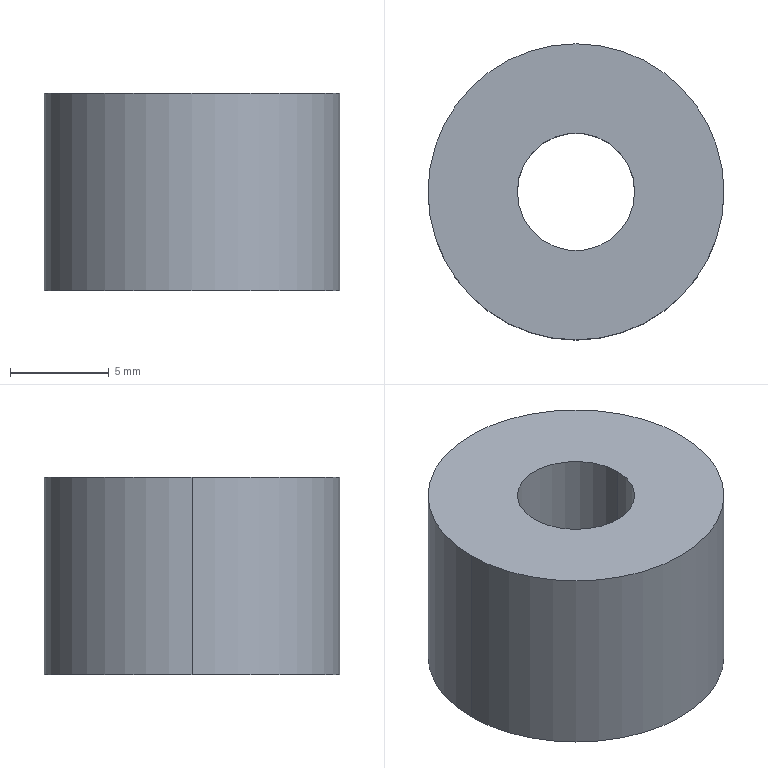Component | SolidWorks | SmallWheel-1 | 1 solid | 6 faces | box 15 x 15 x 10 mm | volume 1489 mm3 | cylinder 4 | plane 2 | commonest cylinder face diameters 5.952 x2 15 x2
build123d program:
from build123d import *

# Parameters (mm, degrees)
SKETCH1_R           = 7.5
SKETCH1_R_2         = 2.976
BOSS_EXTRUDE1_DEPTH = 10


with BuildPart() as part:
    # Sketch1 → Boss-Extrude1 (new body)
    with BuildSketch(Plane.XY):
        with Locations((59.88, -20)):
            Circle(SKETCH1_R)
        with Locations((59.88, -20)):
            Circle(SKETCH1_R_2, mode=Mode.SUBTRACT)
    extrude(amount=-BOSS_EXTRUDE1_DEPTH)


solid = part.part

# Placed as in the assembly
solid = solid.moved(Location((-11.374, -44.609, -195), (0, 0, 0)))
STEP:
#1=COLOUR_RGB('',0.7922,0.8196,0.9333);
#2=FILL_AREA_STYLE_COLOUR('',#1);
#3=FILL_AREA_STYLE('',(#2));
#4=SURFACE_STYLE_FILL_AREA(#3);
#5=SURFACE_SIDE_STYLE('',(#4));
#6=SURFACE_STYLE_USAGE(.BOTH.,#5);
#7=PRESENTATION_STYLE_ASSIGNMENT((#6));
#8=CARTESIAN_POINT('',(1.793,-2.544,-8.071));
#9=VERTEX_POINT('',#8);
#10=CARTESIAN_POINT('',(2.027,-2.544,-8.071));
#11=VERTEX_POINT('',#10);
#12=CARTESIAN_POINT('',(1.91,-2.544,-8.071));
#13=DIRECTION('',(0.,0.,1.));
#14=DIRECTION('',(1.,0.,0.));
#15=AXIS2_PLACEMENT_3D('',#12,#13,#14);
#16=CIRCLE('',#15,0.1172);
#17=EDGE_CURVE('',#9,#11,#16,.T.);
#18=ORIENTED_EDGE('',*,*,#17,.F.);
#19=CARTESIAN_POINT('',(1.793,-2.544,-7.677));
#20=VERTEX_POINT('',#19);
#21=CARTESIAN_POINT('',(1.793,-2.544,-8.071));
#22=DIRECTION('',(0.,0.,1.));
#23=VECTOR('',#22,39.37);
#24=LINE('',#21,#23);
#25=EDGE_CURVE('',#9,#20,#24,.T.);
#26=ORIENTED_EDGE('',*,*,#25,.T.);
#27=CARTESIAN_POINT('',(2.027,-2.544,-7.677));
#28=VERTEX_POINT('',#27);
#29=CARTESIAN_POINT('',(1.91,-2.544,-7.677));
#30=DIRECTION('',(0.,0.,1.));
#31=DIRECTION('',(1.,0.,0.));
#32=AXIS2_PLACEMENT_3D('',#29,#30,#31);
#33=CIRCLE('',#32,0.1172);
#34=EDGE_CURVE('',#20,#28,#33,.T.);
#35=ORIENTED_EDGE('',*,*,#34,.T.);
#36=CARTESIAN_POINT('',(2.027,-2.544,-8.071));
#37=DIRECTION('',(0.,0.,1.));
#38=VECTOR('',#37,39.37);
#39=LINE('',#36,#38);
#40=EDGE_CURVE('',#11,#28,#39,.T.);
#41=ORIENTED_EDGE('',*,*,#40,.F.);
#42=EDGE_LOOP('',(#18,#26,#35,#41));
#43=FACE_OUTER_BOUND('',#42,.T.);
#44=CARTESIAN_POINT('',(1.91,-2.544,-8.071));
#45=DIRECTION('',(0.,0.,1.));
#46=DIRECTION('',(1.,0.,0.));
#47=AXIS2_PLACEMENT_3D('',#44,#45,#46);
#48=CYLINDRICAL_SURFACE('',#47,0.1172);
#49=ADVANCED_FACE('',(#43),#48,.F.);
#50=CARTESIAN_POINT('',(2.205,-2.544,-8.071));
#51=VERTEX_POINT('',#50);
#52=CARTESIAN_POINT('',(1.614,-2.544,-8.071));
#53=VERTEX_POINT('',#52);
#54=CARTESIAN_POINT('',(1.91,-2.544,-8.071));
#55=DIRECTION('',(0.,0.,1.));
#56=DIRECTION('',(1.,0.,0.));
#57=AXIS2_PLACEMENT_3D('',#54,#55,#56);
#58=CIRCLE('',#57,0.2953);
#59=EDGE_CURVE('',#51,#53,#58,.T.);
#60=ORIENTED_EDGE('',*,*,#59,.T.);
#61=CARTESIAN_POINT('',(1.614,-2.544,-7.677));
#62=VERTEX_POINT('',#61);
#63=CARTESIAN_POINT('',(1.614,-2.544,-8.071));
#64=DIRECTION('',(0.,0.,1.));
#65=VECTOR('',#64,39.37);
#66=LINE('',#63,#65);
#67=EDGE_CURVE('',#53,#62,#66,.T.);
#68=ORIENTED_EDGE('',*,*,#67,.T.);
#69=CARTESIAN_POINT('',(2.205,-2.544,-7.677));
#70=VERTEX_POINT('',#69);
#71=CARTESIAN_POINT('',(1.91,-2.544,-7.677));
#72=DIRECTION('',(0.,0.,1.));
#73=DIRECTION('',(1.,0.,0.));
#74=AXIS2_PLACEMENT_3D('',#71,#72,#73);
#75=CIRCLE('',#74,0.2953);
#76=EDGE_CURVE('',#70,#62,#75,.T.);
#77=ORIENTED_EDGE('',*,*,#76,.F.);
#78=CARTESIAN_POINT('',(2.205,-2.544,-8.071));
#79=DIRECTION('',(0.,0.,1.));
#80=VECTOR('',#79,39.37);
#81=LINE('',#78,#80);
#82=EDGE_CURVE('',#51,#70,#81,.T.);
#83=ORIENTED_EDGE('',*,*,#82,.F.);
#84=EDGE_LOOP('',(#60,#68,#77,#83));
#85=FACE_OUTER_BOUND('',#84,.T.);
#86=CARTESIAN_POINT('',(1.91,-2.544,-8.071));
#87=DIRECTION('',(0.,0.,1.));
#88=DIRECTION('',(1.,0.,0.));
#89=AXIS2_PLACEMENT_3D('',#86,#87,#88);
#90=CYLINDRICAL_SURFACE('',#89,0.2953);
#91=ADVANCED_FACE('',(#85),#90,.T.);
#92=ORIENTED_EDGE('',*,*,#67,.F.);
#93=CARTESIAN_POINT('',(1.91,-2.544,-8.071));
#94=DIRECTION('',(0.,0.,1.));
#95=DIRECTION('',(1.,0.,0.));
#96=AXIS2_PLACEMENT_3D('',#93,#94,#95);
#97=CIRCLE('',#96,0.2953);
#98=EDGE_CURVE('',#53,#51,#97,.T.);
#99=ORIENTED_EDGE('',*,*,#98,.T.);
#100=ORIENTED_EDGE('',*,*,#82,.T.);
#101=CARTESIAN_POINT('',(1.91,-2.544,-7.677));
#102=DIRECTION('',(0.,0.,1.));
#103=DIRECTION('',(1.,0.,0.));
#104=AXIS2_PLACEMENT_3D('',#101,#102,#103);
#105=CIRCLE('',#104,0.2953);
#106=EDGE_CURVE('',#62,#70,#105,.T.);
#107=ORIENTED_EDGE('',*,*,#106,.F.);
#108=EDGE_LOOP('',(#92,#99,#100,#107));
#109=FACE_OUTER_BOUND('',#108,.T.);
#110=CARTESIAN_POINT('',(1.91,-2.544,-8.071));
#111=DIRECTION('',(0.,0.,1.));
#112=DIRECTION('',(1.,0.,0.));
#113=AXIS2_PLACEMENT_3D('',#110,#111,#112);
#114=CYLINDRICAL_SURFACE('',#113,0.2953);
#115=ADVANCED_FACE('',(#109),#114,.T.);
#116=CARTESIAN_POINT('',(1.91,-2.544,-8.071));
#117=DIRECTION('',(0.,0.,1.));
#118=DIRECTION('',(1.,0.,0.));
#119=AXIS2_PLACEMENT_3D('',#116,#117,#118);
#120=CIRCLE('',#119,0.1172);
#121=EDGE_CURVE('',#11,#9,#120,.T.);
#122=ORIENTED_EDGE('',*,*,#121,.T.);
#123=ORIENTED_EDGE('',*,*,#17,.T.);
#124=EDGE_LOOP('',(#122,#123));
#125=FACE_BOUND('',#124,.T.);
#126=ORIENTED_EDGE('',*,*,#59,.F.);
#127=ORIENTED_EDGE('',*,*,#98,.F.);
#128=EDGE_LOOP('',(#126,#127));
#129=FACE_OUTER_BOUND('',#128,.T.);
#130=CARTESIAN_POINT('',(1.91,-2.544,-8.071));
#131=DIRECTION('',(0.,0.,1.));
#132=DIRECTION('',(1.,0.,0.));
#133=AXIS2_PLACEMENT_3D('',#130,#131,#132);
#134=PLANE('',#133);
#135=ADVANCED_FACE('',(#125,#129),#134,.F.);
#136=CARTESIAN_POINT('',(1.91,-2.544,-7.677));
#137=DIRECTION('',(0.,0.,1.));
#138=DIRECTION('',(1.,0.,0.));
#139=AXIS2_PLACEMENT_3D('',#136,#137,#138);
#140=CIRCLE('',#139,0.1172);
#141=EDGE_CURVE('',#28,#20,#140,.T.);
#142=ORIENTED_EDGE('',*,*,#141,.F.);
#143=ORIENTED_EDGE('',*,*,#34,.F.);
#144=EDGE_LOOP('',(#142,#143));
#145=FACE_BOUND('',#144,.T.);
#146=ORIENTED_EDGE('',*,*,#76,.T.);
#147=ORIENTED_EDGE('',*,*,#106,.T.);
#148=EDGE_LOOP('',(#146,#147));
#149=FACE_OUTER_BOUND('',#148,.T.);
#150=CARTESIAN_POINT('',(1.91,-2.544,-7.677));
#151=DIRECTION('',(0.,0.,1.));
#152=DIRECTION('',(1.,0.,0.));
#153=AXIS2_PLACEMENT_3D('',#150,#151,#152);
#154=PLANE('',#153);
#155=ADVANCED_FACE('',(#145,#149),#154,.T.);
#156=ORIENTED_EDGE('',*,*,#25,.F.);
#157=ORIENTED_EDGE('',*,*,#121,.F.);
#158=ORIENTED_EDGE('',*,*,#40,.T.);
#159=ORIENTED_EDGE('',*,*,#141,.T.);
#160=EDGE_LOOP('',(#156,#157,#158,#159));
#161=FACE_OUTER_BOUND('',#160,.T.);
#162=CARTESIAN_POINT('',(1.91,-2.544,-8.071));
#163=DIRECTION('',(0.,0.,1.));
#164=DIRECTION('',(1.,0.,0.));
#165=AXIS2_PLACEMENT_3D('',#162,#163,#164);
#166=CYLINDRICAL_SURFACE('',#165,0.1172);
#167=ADVANCED_FACE('',(#161),#166,.F.);
#168=CLOSED_SHELL('',(#49,#91,#115,#135,#155,#167));
#169=MANIFOLD_SOLID_BREP('',#168);
#170=STYLED_ITEM('',(#7),#169);
#171=(LENGTH_UNIT()NAMED_UNIT(*)SI_UNIT($,.METRE.));
#172=LENGTH_MEASURE_WITH_UNIT(LENGTH_MEASURE(0.0254),#171);
#173=DIMENSIONAL_EXPONENTS(1.,0.,0.,0.,0.,0.,0.);
#174=(CONVERSION_BASED_UNIT('',#172)LENGTH_UNIT()NAMED_UNIT(#173));
#175=UNCERTAINTY_MEASURE_WITH_UNIT(LENGTH_MEASURE(0.00001),#174,'','');
#176=(NAMED_UNIT(*)PLANE_ANGLE_UNIT()SI_UNIT($,.RADIAN.));
#177=(NAMED_UNIT(*)SI_UNIT($,.STERADIAN.)SOLID_ANGLE_UNIT());
#178=(GEOMETRIC_REPRESENTATION_CONTEXT(3)GLOBAL_UNCERTAINTY_ASSIGNED_CONTEXT((#175))GLOBAL_UNIT_ASSIGNED_CONTEXT((#174,#176,#177))REPRESENTATION_CONTEXT('',''));
#179=MECHANICAL_DESIGN_GEOMETRIC_PRESENTATION_REPRESENTATION('',(#170),#178);
#180=CARTESIAN_POINT('',(0.,0.,0.));
#181=DIRECTION('',(0.,0.,1.));
#182=DIRECTION('',(1.,0.,0.));
#183=AXIS2_PLACEMENT_3D('',#180,#181,#182);
#184=(LENGTH_UNIT()NAMED_UNIT(*)SI_UNIT($,.METRE.));
#185=LENGTH_MEASURE_WITH_UNIT(LENGTH_MEASURE(0.0254),#184);
#186=DIMENSIONAL_EXPONENTS(1.,0.,0.,0.,0.,0.,0.);
#187=(CONVERSION_BASED_UNIT('',#185)LENGTH_UNIT()NAMED_UNIT(#186));
#188=UNCERTAINTY_MEASURE_WITH_UNIT(LENGTH_MEASURE(0.00001),#187,'','');
#189=(NAMED_UNIT(*)PLANE_ANGLE_UNIT()SI_UNIT($,.RADIAN.));
#190=(NAMED_UNIT(*)SI_UNIT($,.STERADIAN.)SOLID_ANGLE_UNIT());
#191=(GEOMETRIC_REPRESENTATION_CONTEXT(3)GLOBAL_UNCERTAINTY_ASSIGNED_CONTEXT((#188))GLOBAL_UNIT_ASSIGNED_CONTEXT((#187,#189,#190))REPRESENTATION_CONTEXT('',''));
#192=ADVANCED_BREP_SHAPE_REPRESENTATION('',(#169,#183),#191);
#193=PRESENTATION_LAYER_ASSIGNMENT('','',(#170));